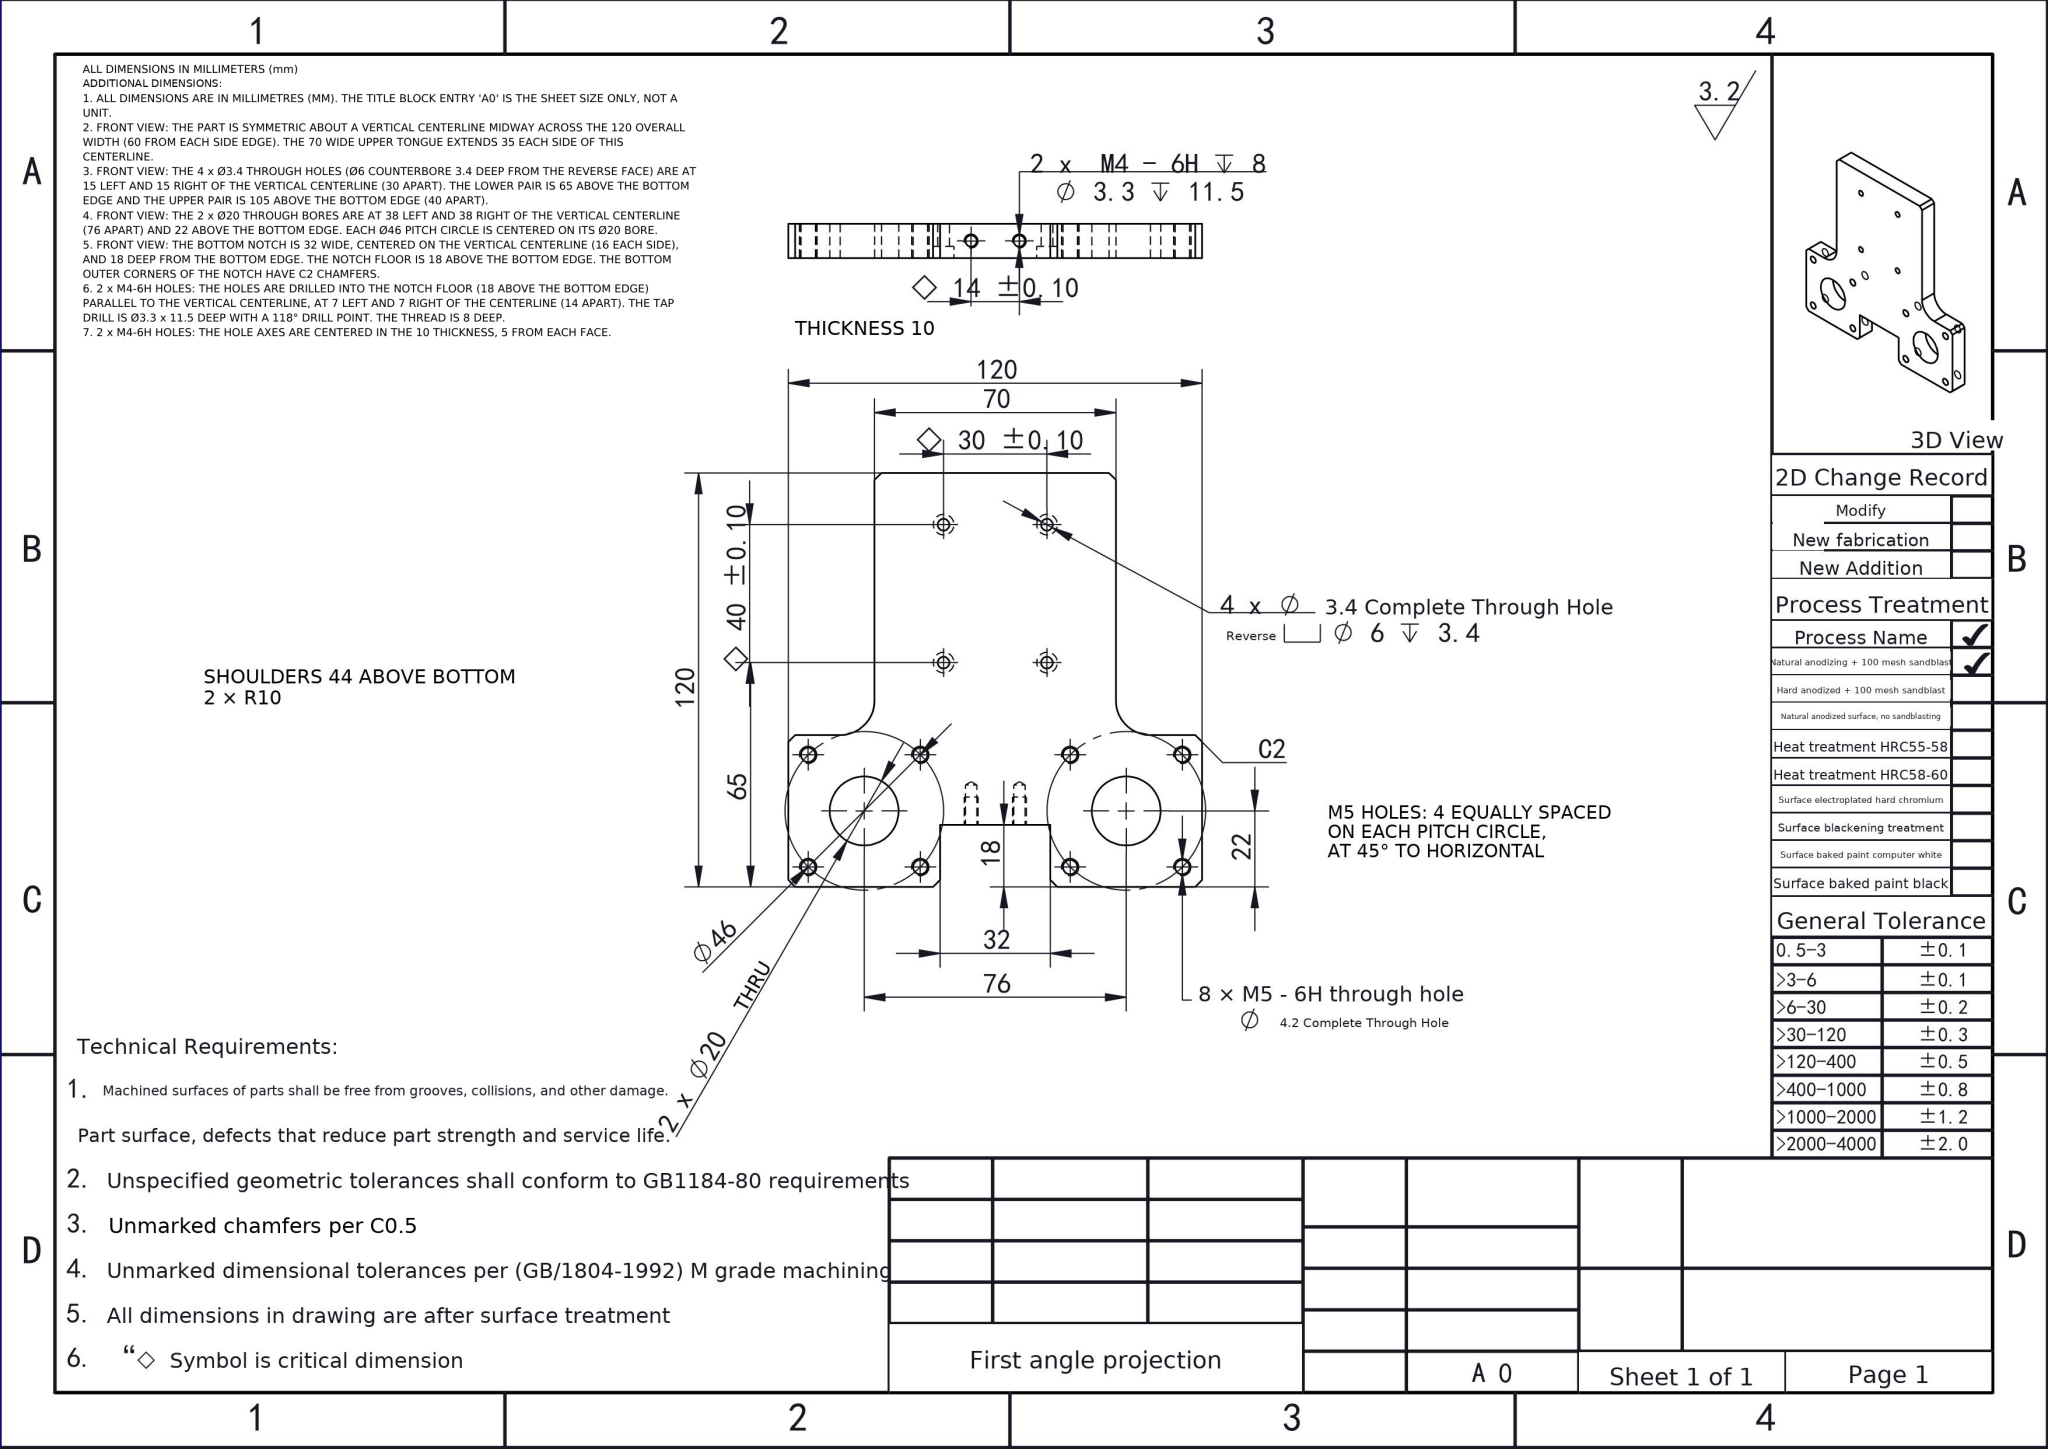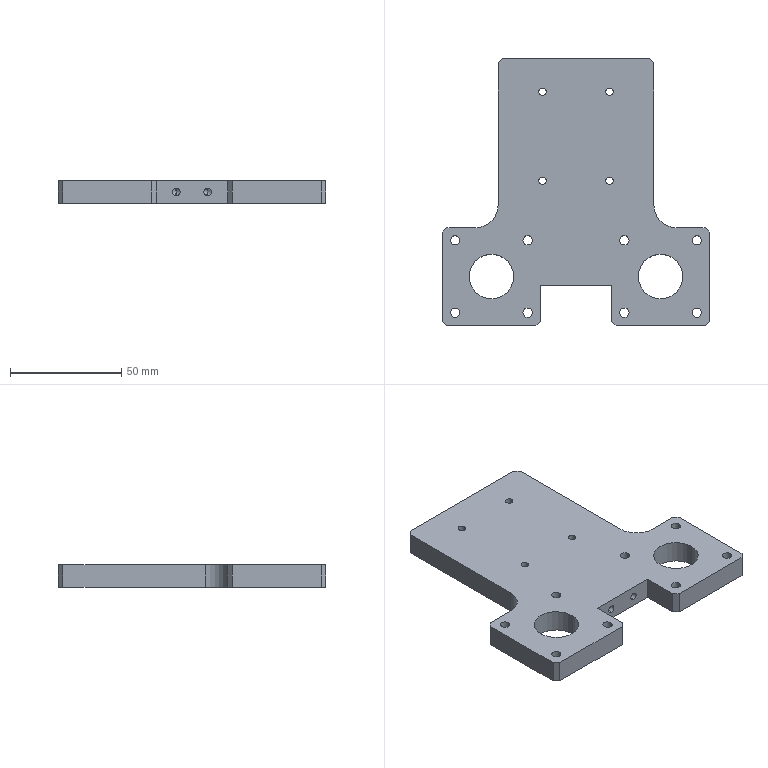Part | NX | mm | 1 solid | 72 faces | box 120 x 120 x 10 mm | volume 92291 mm3 | cylinder 42 | plane 26 | cone 4 | commonest cylinder face diameters 4.2 x16 6 x8 3.4 x8 20 x6 3.3 x4